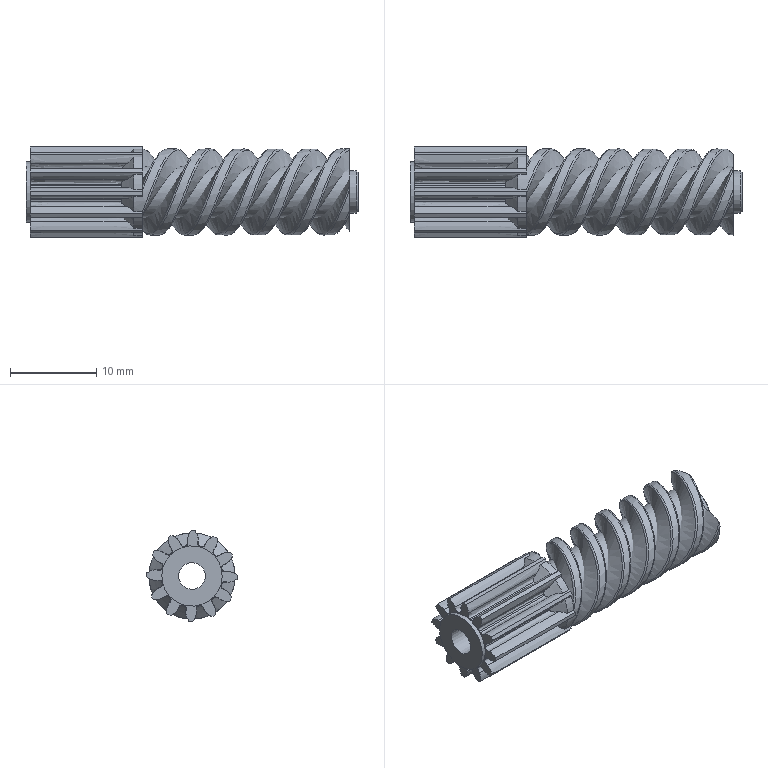Component | NX | DJZ_11_THREADED_SHAFT_LH_2 | 1 solid | 120 faces | volume 1827 mm3 | other 60 | cylinder 27 | cone 14 | spline 12 | plane 7 | commonest cylinder face diameters 10 x12 7.125 x12 4.9 x1 7 x1 3.1 x1